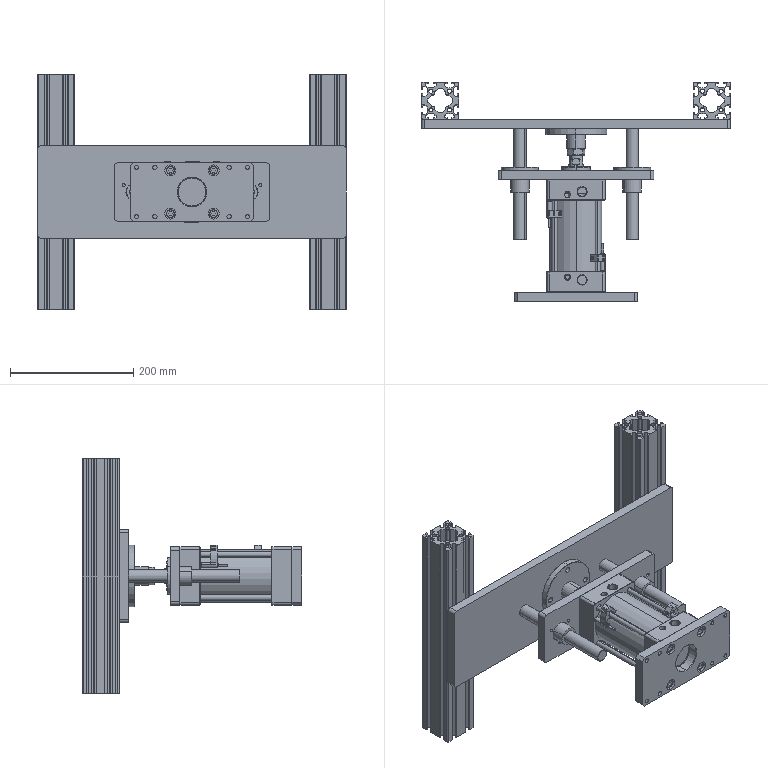Assembly | SolidWorks | mm | 27 component files | 27 solids | 1656 faces | box 500 x 356 x 380 mm | volume 3765286 mm3 | plane 796 | cylinder 523 | cone 191 | torus 146 | commonest cylinder face diameters 10 x40 0.6 x36 2 x36 8 x33 7 x31 6.8 x28 6 x24 16 x21
Bill of materials:
FCS1_A_SC80 | 2 |  | Clamp- or gripper-like body: two curved jaw arms with stepped/toothed inner faces, coming off a cylindrical barrel, with a smaller stepped round shaft sticking out of one end of the barrel.
FJSI80_3 | 4 |  | Hollow cylindrical sleeve with rounded/chamfered end edges. One end shows a hexagonal internal recess and the other end shows a round bore.
FSC_80_Screw | 4 | Plain Carbon Steel | Stepped cylindrical pin shaped like a socket-head cap screw: a larger cylindrical head with a hexagonal socket recess, and a smaller plain cylindrical shank with a chamfered tip.
FSC_80x75_S_FB_0_c | 1 |  | Cylindrical tube body held between two square end blocks, with a short round boss sticking out of one end. The end face has four corner through holes, a central circular boss, and radiating slots/grooves.
FSC80_753 | 4 |  | Long slender round rod with a larger-diameter cylindrical end section at one end and a short, slightly larger stepped end section at the other.
FSC_80_M20x1_5_Nut | 1 |  | Hexagonal nut-like ring: a hex prism with chamfered corners on both faces and a plain circular through bore.
FSC_80x75_S_FB_0_r | 1 |  | Axially symmetric shaft-like body: a hollow front spigot, a wider hub with several circumferential grooves and ribs held by radial spokes, and a long stepped shaft with a flat or reduced section near the end.
E000-HFSG6_6060_380 | 2 |  | Straight prismatic bar with a constant square cross-section, shaped like a slotted structural extrusion profile. Each of the four sides has two T-shaped slots running the full length (eight slots in total). The section has a large central octagonal cavity, four round through-bores parallel to the length (one near each corner), rounded outer corners, and webs running diagonally from the core to the corners.
E001CylinderRearFlangePlate | 1 | Plain Carbon Steel | Flat rectangular plate with chamfered corners, a large central through hole, four medium through holes arranged around the center, and eight small through holes near the edges.
E002GuidePlate | 1 | Plain Carbon Steel | Flat rectangular plate with rounded corners: a large central hole, two medium holes on either side each surrounded by three small holes, and four medium holes around the central hole.
E003CopperSleeve | 2 | Brass | Flanged bushing: a round flange with three through holes evenly spaced on a circle, and a cylindrical hub sticking out with a central through bore.
E004Tray | 1 | Plain Carbon Steel | Round flange with four through holes evenly spaced on a circle and a short cylindrical hub on one side with a central through bore.
E005GuideAxis | 2 | Stainless Steel (Ferritic) | Plain solid cylindrical rod with a short reduced-diameter step at one end.
E006TopPlate | 1 | Plain Carbon Steel | Thin, flat rectangular plate with small rounded corners and six through holes. The holes sit symmetrically about the plate center: two larger holes on the long centerline, two smaller holes on the same line between them, and two smaller holes on the short centerline above and below center. The four small holes form a diamond pattern.
Mates:
1. coincident | assembly face at (100, 0, -47.5) dir (0, -1, 0) | assembly plane at (0, 0, 0) dir (0, 1, 0)
2. coincident | AirTACCylinderFSC_80x75_S_FB-1 plane at (0, 198, 0) dir (1, 0, 0) | assembly plane at (0, 0, 0) dir (1, 0, 0)
3. coincident | AirTACCylinderFSC_80x75_S_FB-1 plane at (0, 198, 0) dir (0, 0, 1) | assembly plane at (0, 0, 0) dir (0, 0, 1)
4. concentric | E002GuidePlate-1 face at (91, 198, 0) dir (0, 1, 0) r 16 | E003CopperSleeve-1 face at (91, 218, 0) dir (0, 1, 0) r 15
5. coincident | E002GuidePlate-1 face at (126, 213, 47) dir (0, 1, 0) | E003CopperSleeve-1 face at (83.5, 213, -12.99) dir (0, -1, 0)
6. concentric | E002GuidePlate-1 face at (91, 213, -22.5) dir (0, 1, 0) r 2.5 | E003CopperSleeve-1 face at (91, 178, -22.5) dir (0, 1, 0) r 3.5
7. concentric | E002GuidePlate-1 face at (-91, 198, 0) dir (0, 1, 0) r 16 | E003CopperSleeve-2 face at (-91, 218, 0) dir (0, 1, 0) r 10
8. concentric | E002GuidePlate-1 face at (-91, 213, -22.5) dir (0, 1, 0) r 2.5 | E003CopperSleeve-2 face at (-91, 178, -22.5) dir (0, 1, 0) r 3.5
9. coincident | E002GuidePlate-1 face at (126, 213, 47) dir (0, 1, 0) | E003CopperSleeve-2 face at (-98.5, 213, -12.99) dir (0, -1, 0)
10. concentric | E005GuideAxis-1 face at (-91, 296, 0) dir (0, -1, 0) r 10 | E003CopperSleeve-2 face at (-91, 218, 0) dir (0, 1, 0) r 10
11. concentric | assembly face at (0, 19, 0) dir (0, 1, 0) r 10 | E004Tray-1 face at (0, 248, 0) dir (0, -1, 0) r 8.75
12. coincident | assembly face at (0, 248, 0) dir (0, 1, 0) | E004Tray-1 face at (0, 248, 0) dir (0, -1, 0)
13. coincident | E004Tray-1 face at (-49.999, 281, -0.35) dir (0, 1, 0) | E006TopPlate-1 face at (250, 281, 75) dir (0, -1, 0)
14. concentric | E006TopPlate-1 face at (-91, 281, 0) dir (0, 1, 0) r 7.5 | E005GuideAxis-1 face at (-91, 296, 0) dir (0, -1, 0) r 10
15. concentric | E003CopperSleeve-1 face at (91, 218, 0) dir (0, 1, 0) r 10 | E005GuideAxis-2 face at (91, 296, 0) dir (0, -1, 0) r 10
16. coincident | E005GuideAxis-1 face at (-91, 101, 0) dir (0, -1, 0) | E005GuideAxis-2 face at (91, 101, 0) dir (0, -1, 0)
17. coincident | E006TopPlate-1 face at (250, 296, 75) dir (0, 1, 0) | E005GuideAxis-2 face at (91, 296, 0) dir (0, 1, 0)
18. concentric | E006TopPlate-1 face at (91, 281, 0) dir (0, 1, 0) r 7.5 | E005GuideAxis-2 face at (91, 296, 0) dir (0, -1, 0) r 10
19. coincident | E006TopPlate-1 face at (250, 296, 75) dir (0, 1, 0) | E000-HFSG6_6060_380-1 face at (209.3, 296, -190) dir (0, -1, 0)
20. coincident | E006TopPlate-1 face at (250, 296, -75) dir (1, 0, 0) | E000-HFSG6_6060_380-1 face at (250, 315.3, -190) dir (1, 0, 0)
21. coincident | E006TopPlate-1 plane at (0, 288.5, 0) dir (0, 0, -1) | E000-HFSG6_6060_380-1 plane at (220, 326, 0) dir (0, 0, 1)
22. coincident | E006TopPlate-1 face at (250, 296, 75) dir (0, 1, 0) | E000-HFSG6_6060_380-2 face at (-209.3, 296, 190) dir (0, -1, 0)
23. coincident | E006TopPlate-1 face at (-250, 296, -75) dir (-1, 0, 0) | E000-HFSG6_6060_380-2 face at (-250, 315.3, 190) dir (-1, 0, 0)
24. coincident | E000-HFSG6_6060_380-1 face at (190.3, 345.3, 190) dir (0, 0, 1) | E000-HFSG6_6060_380-2 face at (-190.3, 345.3, 190) dir (0, 0, 1)
25. concentric | AirTACCylinderFSC_80x75_S_FB-1/FSC_80x75_S_FB_0_c-1 face at (0, 178, 0) dir (0, 1, 0) r 23.5 | E002GuidePlate-1 face at (0, 197.999, 0) dir (0, 1, 0) r 25
26. coincident | AirTACCylinderFSC_80x75_S_FB-1/FSC_80x75_S_FB_0_c-1 face at (43, 198, 43) dir (0, 1, 0) | E002GuidePlate-1 face at (126, 198, 47) dir (0, -1, 0)
27. parallel | AirTACCylinderFSC_80x75_S_FB-1/FSC_80x75_S_FB_0_c-1 face at (43, 165, 47) dir (0, 0, 1) | E002GuidePlate-1 face at (-126, 213, 47) dir (0, 0, 1)
28. concentric | AirTACCylinderFSC_80x75_S_FB-1/FSC_80x75_S_FB_0_c-1 face at (0, 49, 0) dir (0, 1, 0) r 43 | E001CylinderRearFlangePlate-1 face at (0, 0, 0) dir (0, -1, 0) r 23.65
29. coincident | AirTACCylinderFSC_80x75_S_FB-1/FSC_80x75_S_FB_0_c-1 face at (43, 16, 43) dir (0, -1, 0) | E001CylinderRearFlangePlate-1 face at (100, 16, -47.5) dir (0, 1, 0)
30. parallel | AirTACCylinderFSC_80x75_S_FB-1/FSC_80x75_S_FB_0_c-1 face at (43, 49, 47) dir (0, 0, 1) | E001CylinderRearFlangePlate-1 face at (-100, 16, 47.5) dir (0, 0, 1)
31. concentric | AirTACCylinderFSC_80x75_S_FB-1/FSC_80x75_S_FB_0_c-1 face at (0, 49, 0) dir (0, 1, 0) r 43 | AirTACCylinderFSC_80x75_S_FBAxis-1/FSC_80x75_S_FB_0_r-1 face at (0, 19, 0) dir (0, 1, 0) r 12.5
32. coincident | E004Tray-1 face at (0, 248, 0) dir (0, -1, 0) | AirTACCylinderFSC_80x75_S_FBAxis-1/FSC_80_M20x1_5_Nut-1 face at (0, 248, 0) dir (0, 1, 0)
33. coincident | E001CylinderRearFlangePlate-1 face at (100, 0, -47.5) dir (0, -1, 0) | assembly plane at (0, 0, 0) dir (0, 1, 0)
34. distance | AirTACCylinderFSC_80x75_S_FBAxis-1/FSC_80x75_S_FB_0_r-1 face at (0, 273, 0) dir (0, 1, 0) | AirTACCylinderFSC_80x75_S_FB-1/FSC_80x75_S_FB_0_c-1 face at (0, 219, 0) dir (0, 1, 0)
35. distance | FSC_80_M20x1_5_Nut-1 face at (-50, 0, 0) dir (-1, 0, 0) | FSC_80x75_S_FB_0_r-1 face at (-75, 0, 0) dir (-1, 0, 0)
36. concentric | FSC_80x75_S_FB_0_r-1 face at (179, 0, 0) dir (-1, 0, 0) r 10 | FSC_80_M20x1_5_Nut-1 axis at (30.9, 0, 0) dir (-1, 0, 0)